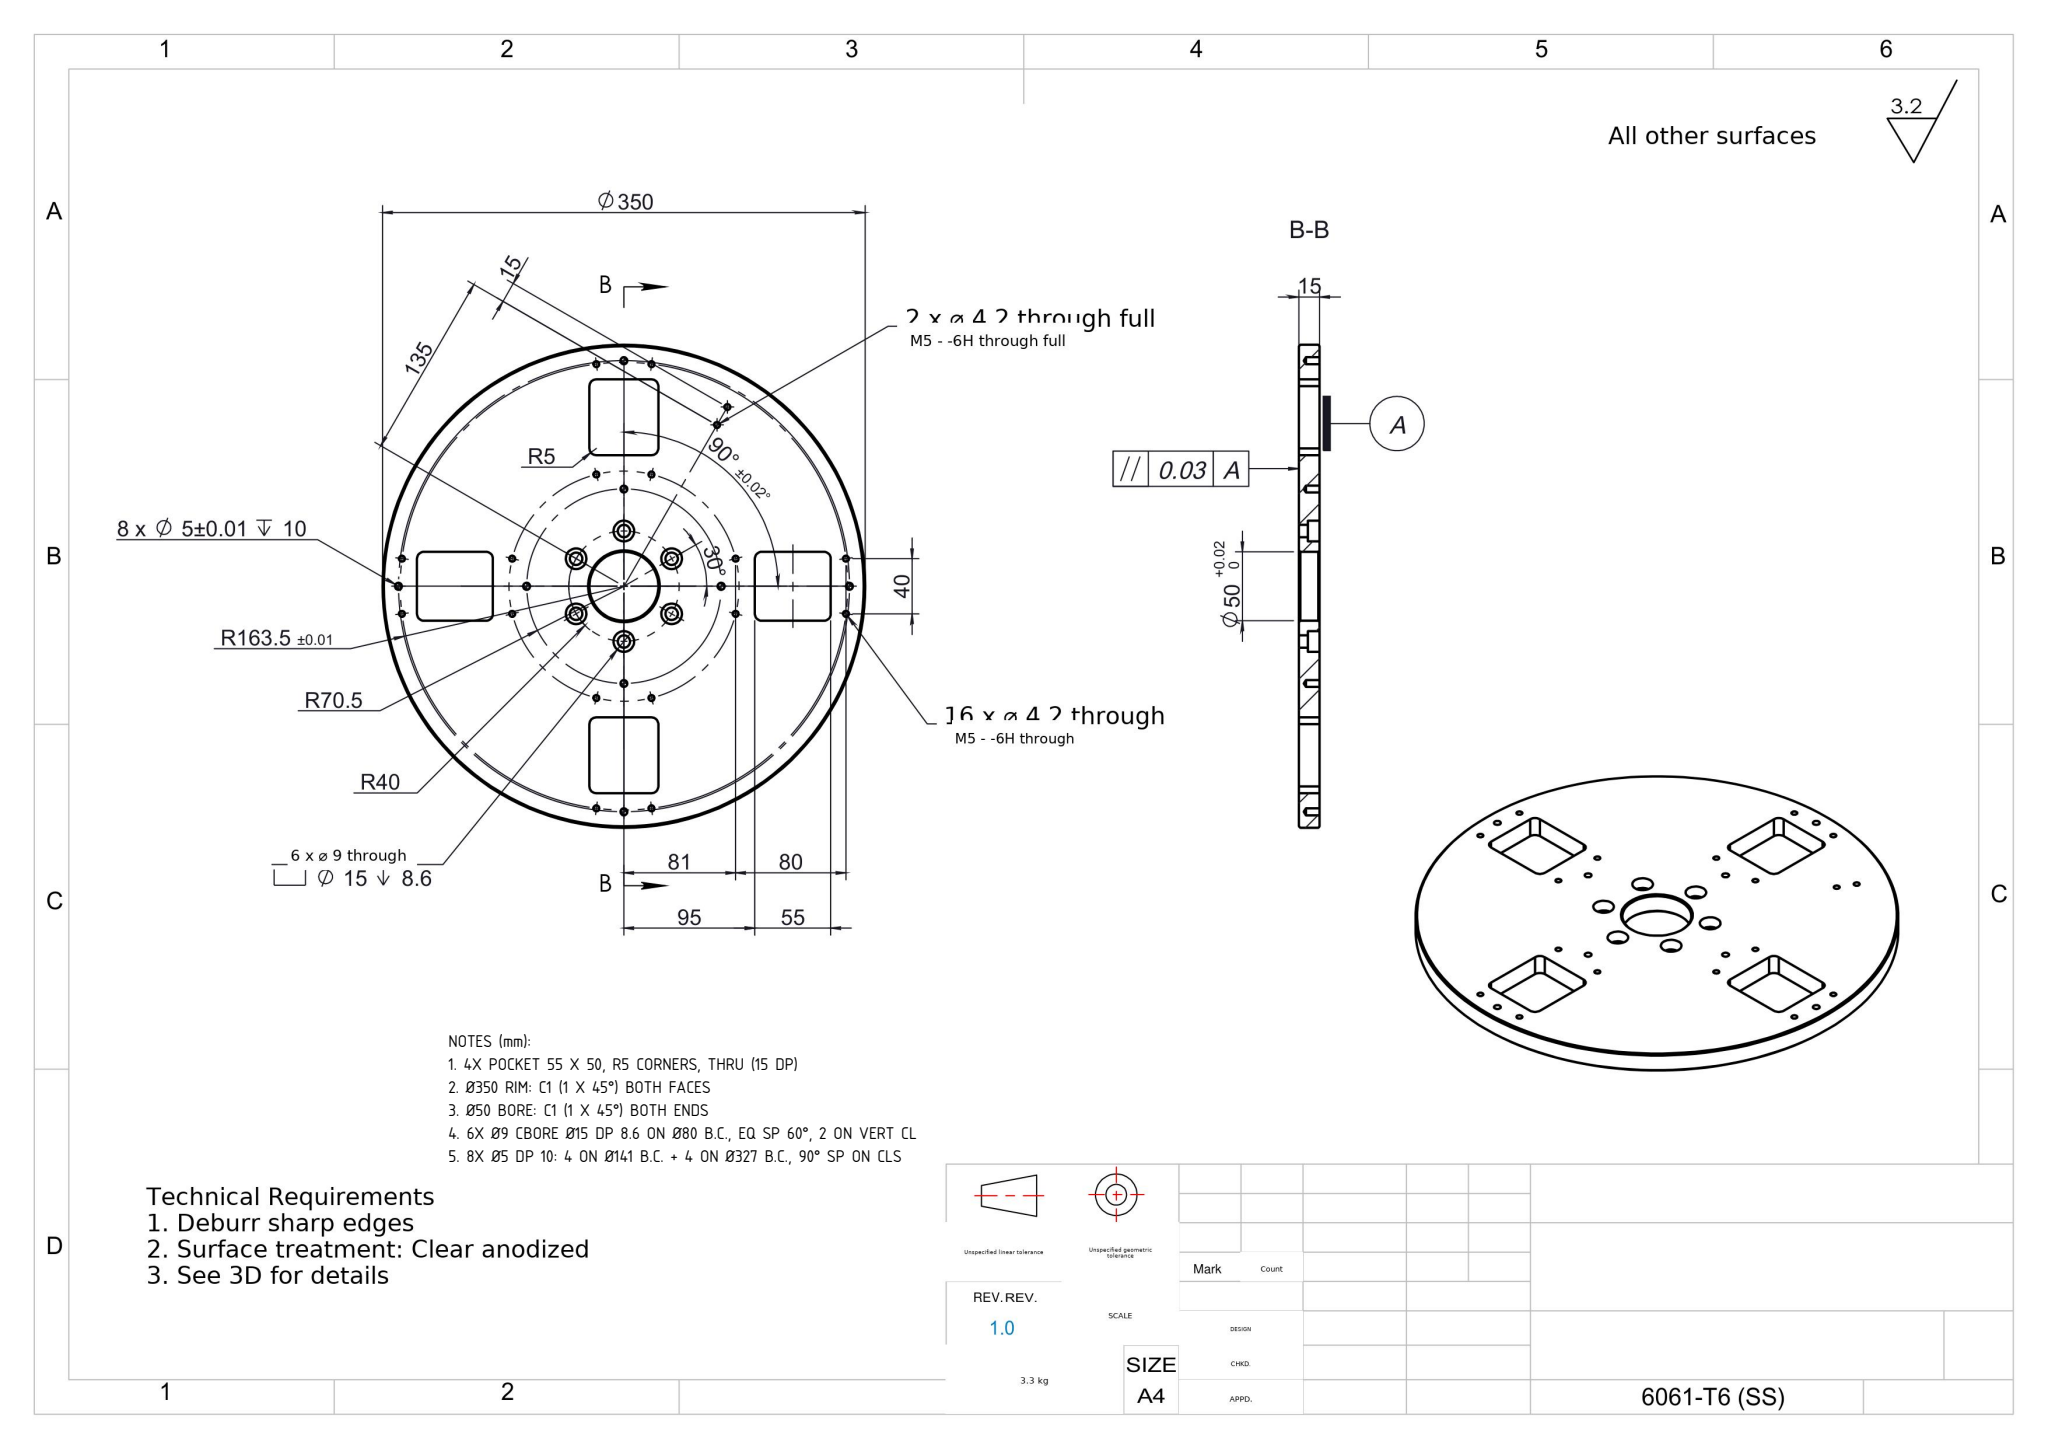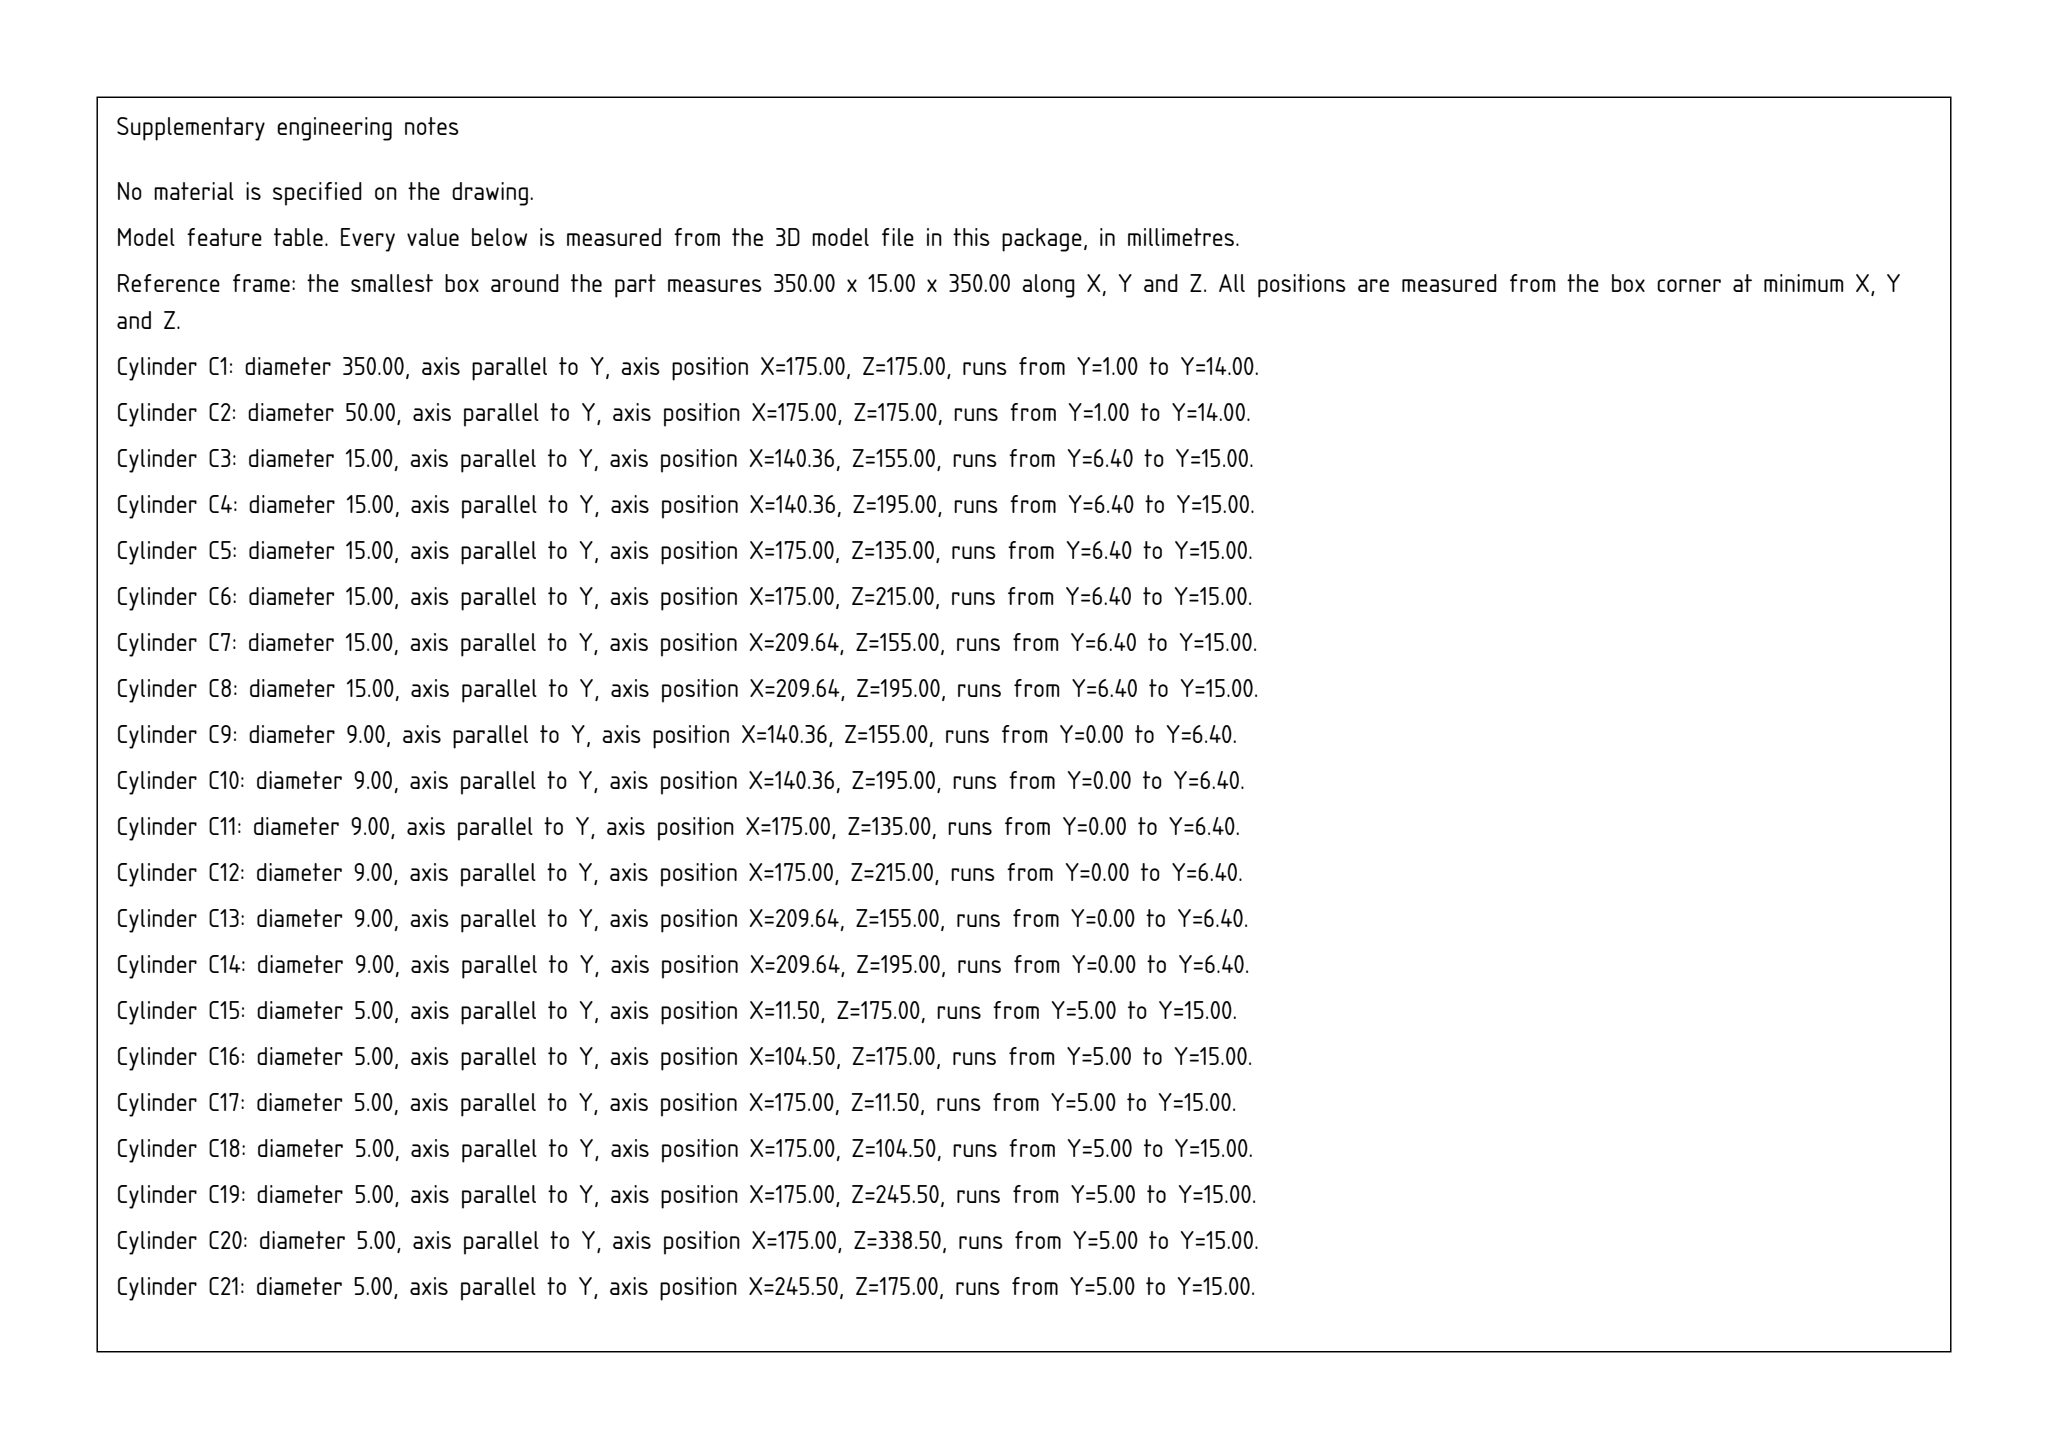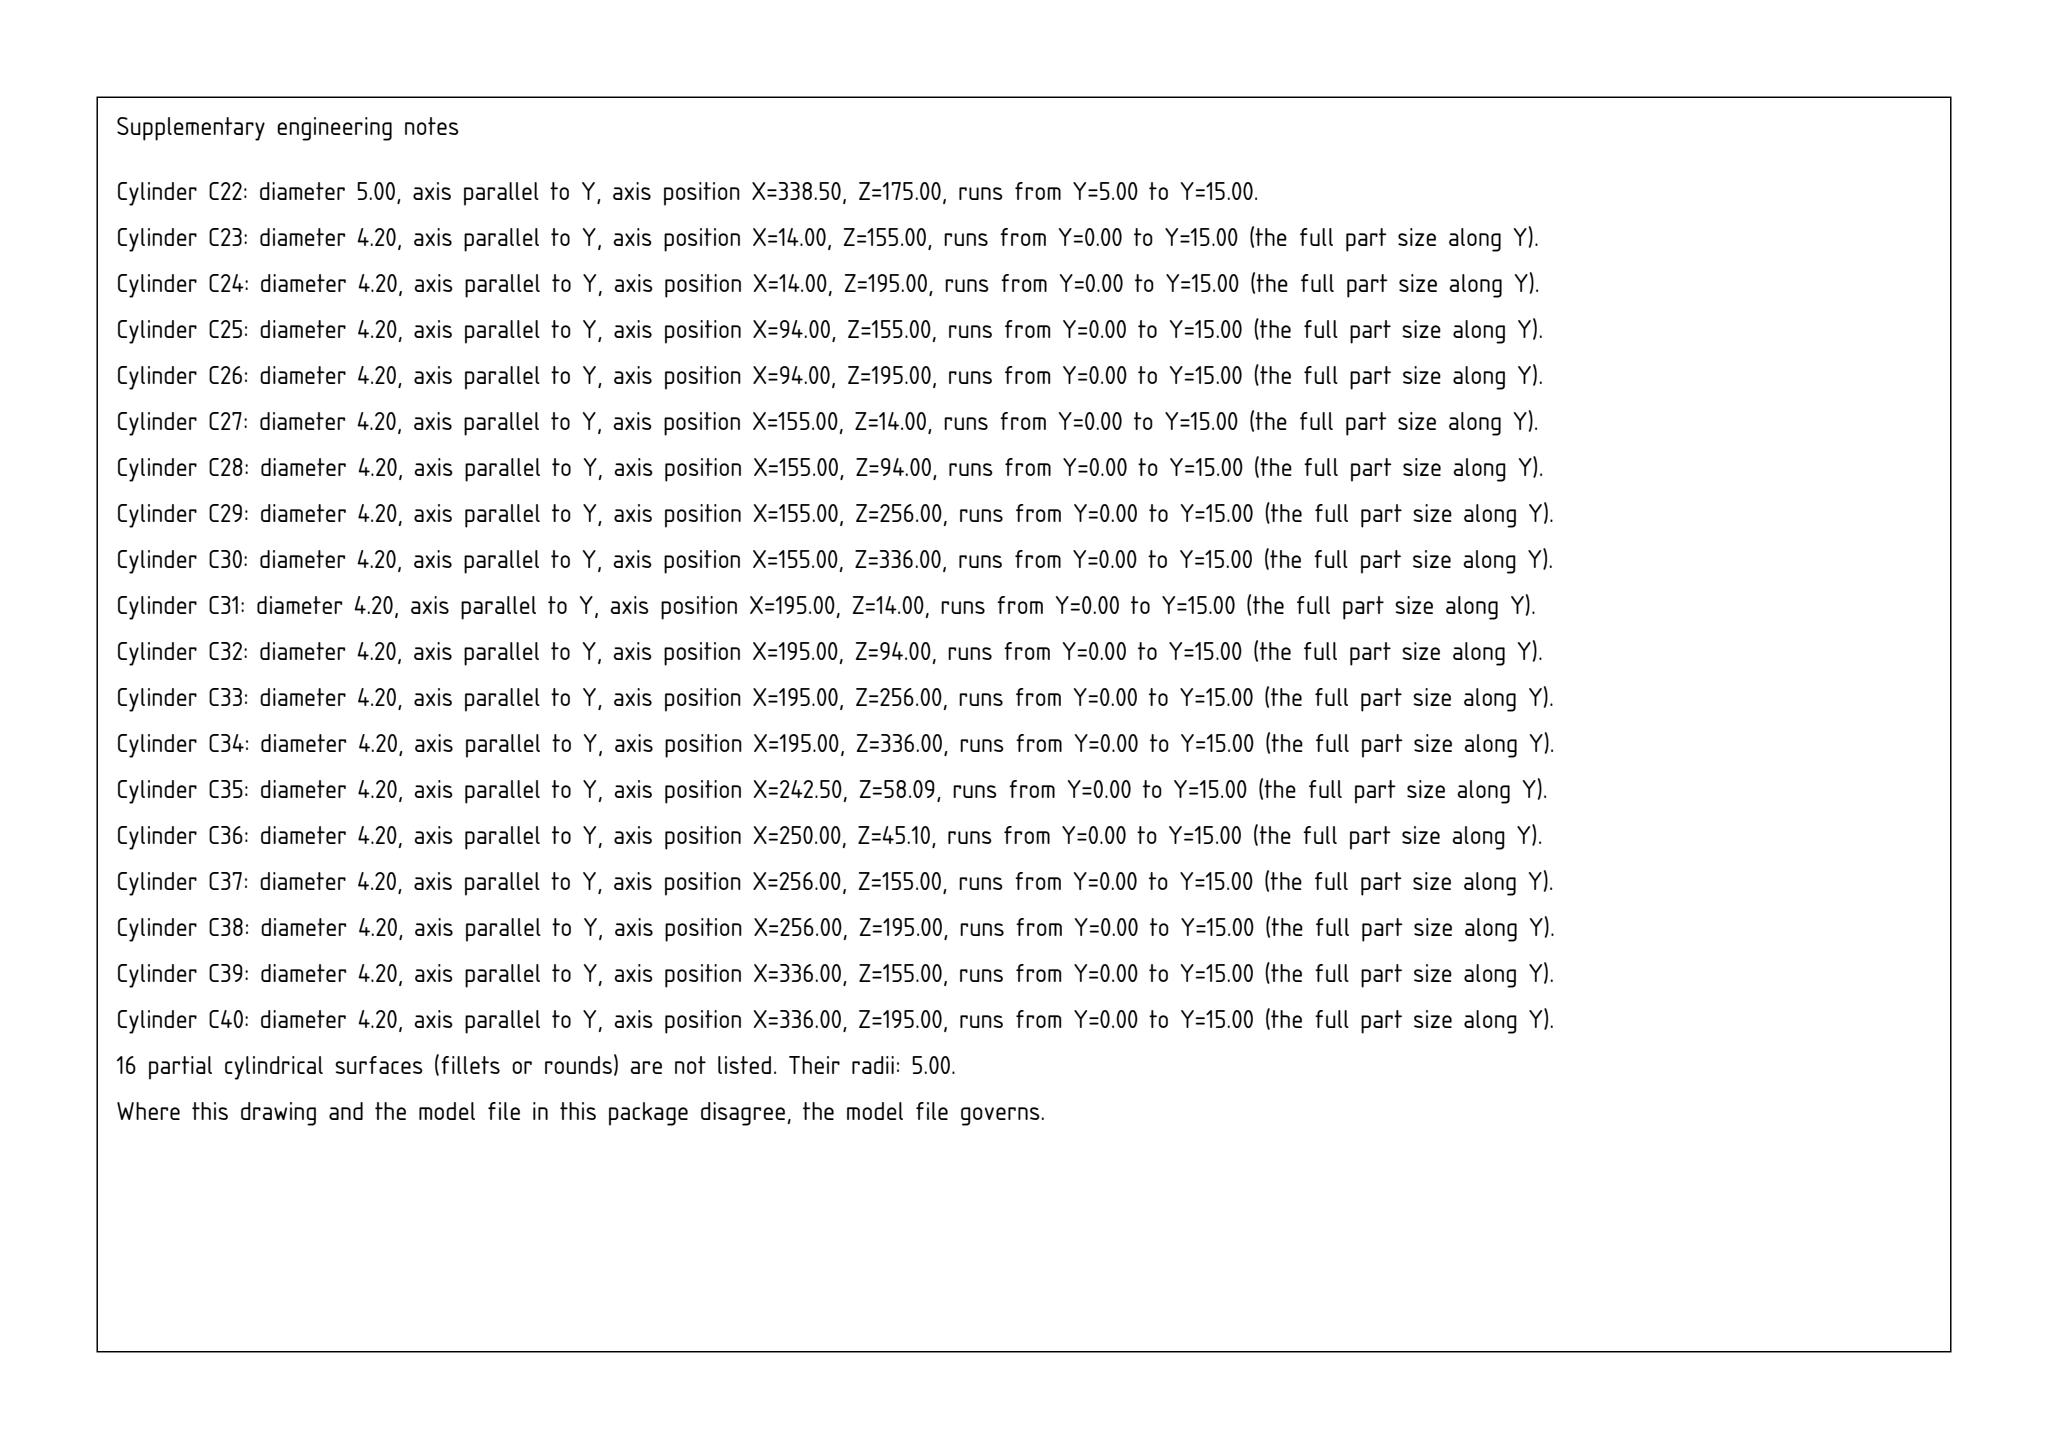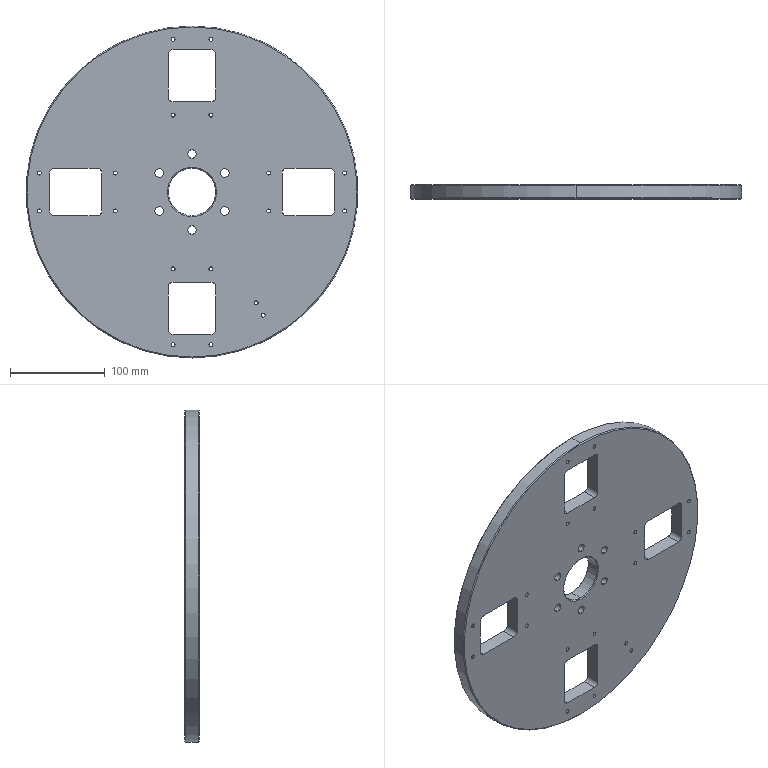Part | SolidWorks | mm | 1 solid | 144 faces | box 350 x 15 x 350 mm | volume 1231796 mm3 | cylinder 96 | cone 24 | plane 24 | commonest cylinder face diameters 4.2 x36 5 x16 10 x16 15 x12 9 x12 50 x2 350 x2
Drawing notes:
4X POCKET 55 X 50, R5 CORNERS, THRU (15 DP) | from the solid: Pocket walls x=25/80 & z=150/200 (55 x 50); R5 corner cyls dia10 L=15 = full plate thk; no floor plane
Ø350 RIM: C1 (1 X 45°) BOTH FACES | from the solid: Cones 90° incl, ref dia 350 & 348 (x2 ea) = 1 mm radial chamfer each face of rim
Ø50 BORE: C1 (1 X 45°) BOTH ENDS | from the solid: Cones 90° incl, ref dia 50 & 52 (x2 ea) at bore Ø50, pos [175,175]
6X Ø9 CBORE Ø15 DP 8.6 ON Ø80 B.C., EQ SP 60°, 2 ON VERT CL | from the solid: Ø9 holes at (140.36,155),(140.36,195),(175,135),(175,215),(209.64,155),(209.64,195) vs ctr (175,175) = R40, 60° sp
8X Ø5 DP 10: 4 ON Ø141 B.C. + 4 ON Ø327 B.C., 90° SP ON CLS | from the solid: Ø5 L=10 holes at r=70.5 (104.5/245.5 on CL) and r=163.5 (11.5/338.5 on CL) from ctr (175,175)
build123d program:
from build123d import *

# Parameters (mm, degrees)
SKETCH1_R                                       = 175
BOSS_EXTRUDE1_DEPTH                             = 15
SKETCH2_R                                       = 25
CUT_EXTRUDE1_DEPTH                              = 248.942
M5_TAPPED_HOLE1_D                               = 4.2
SKETCH5_W                                       = 50
SKETCH5_H                                       = 55
CUT_EXTRUDE2_DEPTH                              = 248.942
FILLET1_R                                       = 5
CIRPATTERN1_COUNT                               = 4
FILLET1_OF_CIRPATTERN1_R                        = 5
M5_TAPPED_HOLE2_D                               = 4.2
CIRPATTERN2_COUNT                               = 4
SIZE_MM_DOWEL_PIN_HOLE_0_AT_2_COUNT             = 2
SIZE_MM_DOWEL_PIN_HOLE_0_AT_2_PITCH             = 93
CIRPATTERN3_COUNT                               = 4
M8_HEX_SOCKET_HEAD_CAP_SCREW_CBORE1_D           = 9
M8_HEX_SOCKET_HEAD_CAP_SCREW_CBORE1_CBORE_D     = 15
M8_HEX_SOCKET_HEAD_CAP_SCREW_CBORE1_CBORE_DEPTH = 8.6
CHAMFER1_SIZE                                   = 1


with BuildPart() as part:
    # Sketch1 → Boss-Extrude1 (new body)
    with BuildSketch(Plane(origin=(0, 0, 0), x_dir=(1, 0, 0), z_dir=(0, 1, 0))):
        with Locations(Location((0, 0, 0), (0, 0, 270))):
            Circle(SKETCH1_R)
    extrude(amount=BOSS_EXTRUDE1_DEPTH)

    # Sketch2 → Cut-Extrude1 (cut, through all)
    with BuildSketch(Plane(origin=(0, 15, 0), x_dir=(1, 0, 0), z_dir=(0, 1, 0))):
        with Locations(Location((0, 0, 0), (0, 0, 270))):
            Circle(SKETCH2_R)
    extrude(amount=-CUT_EXTRUDE1_DEPTH, mode=Mode.SUBTRACT)

    # M5 Tapped Hole1 (through all)
    with Locations(Plane(origin=(0, 15, 0), x_dir=(1, 0, 0), z_dir=(0, 1, 0))):
        with Locations((67.5, 116.913), (75, 129.904)):
            Hole(M5_TAPPED_HOLE1_D / 2)

    # Sketch5 → Cut-Extrude2 (cut, through all)
    with BuildSketch(Plane(origin=(0, 15, 0), x_dir=(1, 0, 0), z_dir=(0, 1, 0))):
        with Locations((0, -122.5)):
            Rectangle(SKETCH5_W, SKETCH5_H)
    cut_extrude2 = extrude(amount=-CUT_EXTRUDE2_DEPTH, mode=Mode.SUBTRACT)

    # Fillet1
    fillet1_edges = [part.edges().sort_by_distance(p)[0] for p in [
        (-25, 7.5, 150),
        (-25, 7.5, 95),
        (25, 7.5, 95),
        (25, 7.5, 150),
    ]]
    fillet(fillet1_edges, radius=FILLET1_R)

    # CirPattern1: Cut-Extrude2 ×4 about axis
    cirpattern1_axis = Axis((0, 0, 0), (0, 1, 0))
    for i in range(1, CIRPATTERN1_COUNT):
        add(cut_extrude2.rotate(cirpattern1_axis, i * 360 / CIRPATTERN1_COUNT), mode=Mode.SUBTRACT)

    # Fillet1 of CirPattern1
    fillet1_of_cirpattern1_edges = [part.edges().sort_by_distance(p)[0] for p in [
        (150, 7.5, 25),
        (95, 7.5, 25),
        (95, 7.5, -25),
        (150, 7.5, -25),
        (25, 7.5, -150),
        (25, 7.5, -95),
        (-25, 7.5, -95),
        (-25, 7.5, -150),
        (-150, 7.5, -25),
        (-95, 7.5, -25),
        (-95, 7.5, 25),
        (-150, 7.5, 25),
    ]]
    fillet(fillet1_of_cirpattern1_edges, radius=FILLET1_OF_CIRPATTERN1_R)

    # M5 Tapped Hole2 (through all)
    with Locations(Plane(origin=(0, 15, 0), x_dir=(1, 0, 0), z_dir=(0, 1, 0))):
        with Locations((20, -81), (-20, -81), (20, -161), (-20, -161)):
            m5_tapped_hole2 = Hole(M5_TAPPED_HOLE2_D / 2)

    # CirPattern2: M5 Tapped Hole2 ×4 about axis
    cirpattern2_axis = Axis((0, 0, 0), (0, 1, 0))
    for i in range(1, CIRPATTERN2_COUNT):
        add(m5_tapped_hole2.rotate(cirpattern2_axis, i * 360 / CIRPATTERN2_COUNT), mode=Mode.SUBTRACT)

    # Sketch9 → Size mm Dowel Pin Hole 0 (revolve, cut)
    with BuildSketch(Plane(origin=(0, 15, 70.5), x_dir=(0, 0, 1), z_dir=(1, 0, 0))):
        Polygon((0, 0), (0, 11.502), (2.5, 10), (2.5, 0), align=None)
    size_mm_dowel_pin_hole_0 = revolve(axis=Axis((0, 21.35, 70.5), (0, -1, 0)), mode=Mode.SUBTRACT)

    # Size mm Dowel Pin Hole 0 at 2: Size mm Dowel Pin Hole 0 ×2
    with Locations(*[(0, 0, i * SIZE_MM_DOWEL_PIN_HOLE_0_AT_2_PITCH) for i in range(1, SIZE_MM_DOWEL_PIN_HOLE_0_AT_2_COUNT)]):
        add(size_mm_dowel_pin_hole_0, mode=Mode.SUBTRACT)

    # CirPattern3: Size mm Dowel Pin Hole 0 ×4 about axis
    cirpattern3_axis = Axis((0, 0, 0), (0, 1, 0))
    for i in range(1, CIRPATTERN3_COUNT):
        add(size_mm_dowel_pin_hole_0.rotate(cirpattern3_axis, i * 360 / CIRPATTERN3_COUNT), mode=Mode.SUBTRACT)

    # CirPattern3 copy 1 sketch → CirPattern3 copy 1 (revolve, cut)
    with BuildSketch(Plane(origin=(163.5, 15, 0), x_dir=(1, 0, 0), z_dir=(0, 0, -1))):
        Polygon((0, 0), (0, 11.502), (2.5, 10), (2.5, 0), align=None)
    revolve(axis=Axis((163.5, 21.35, 0), (0, -1, 0)), mode=Mode.SUBTRACT)

    # CirPattern3 copy 2 sketch → CirPattern3 copy 2 (revolve, cut)
    with BuildSketch(Plane(origin=(0, 15, -163.5), x_dir=(0, 0, -1), z_dir=(-1, 0, 0))):
        Polygon((0, 0), (0, 11.502), (2.5, 10), (2.5, 0), align=None)
    revolve(axis=Axis((0, 21.35, -163.5), (0, -1, 0)), mode=Mode.SUBTRACT)

    # CirPattern3 copy 3 sketch → CirPattern3 copy 3 (revolve, cut)
    with BuildSketch(Plane(origin=(-163.5, 15, 0), x_dir=(-1, 0, 0), z_dir=(0, 0, 1))):
        Polygon((0, 0), (0, 11.502), (2.5, 10), (2.5, 0), align=None)
    revolve(axis=Axis((-163.5, 21.35, 0), (0, -1, 0)), mode=Mode.SUBTRACT)

    # M8 Hex Socket Head Cap Screw CBORE1 (through all)
    with Locations(Plane(origin=(0, 15, 0), x_dir=(1, 0, 0), z_dir=(0, 1, 0))):
        with Locations((0, -40), (-34.641, -20), (-34.641, 20), (0, 40), (34.641, 20), (34.641, -20)):
            CounterBoreHole(M8_HEX_SOCKET_HEAD_CAP_SCREW_CBORE1_D / 2, M8_HEX_SOCKET_HEAD_CAP_SCREW_CBORE1_CBORE_D / 2, M8_HEX_SOCKET_HEAD_CAP_SCREW_CBORE1_CBORE_DEPTH)

    # Chamfer1
    chamfer1_edges = [part.edges().sort_by_distance(p)[0] for p in [
        (0, 0, -25),
        (0, 15, -25),
        (0, 0, -175),
        (0, 15, -175),
    ]]
    chamfer(chamfer1_edges, length=CHAMFER1_SIZE)


solid = part.part